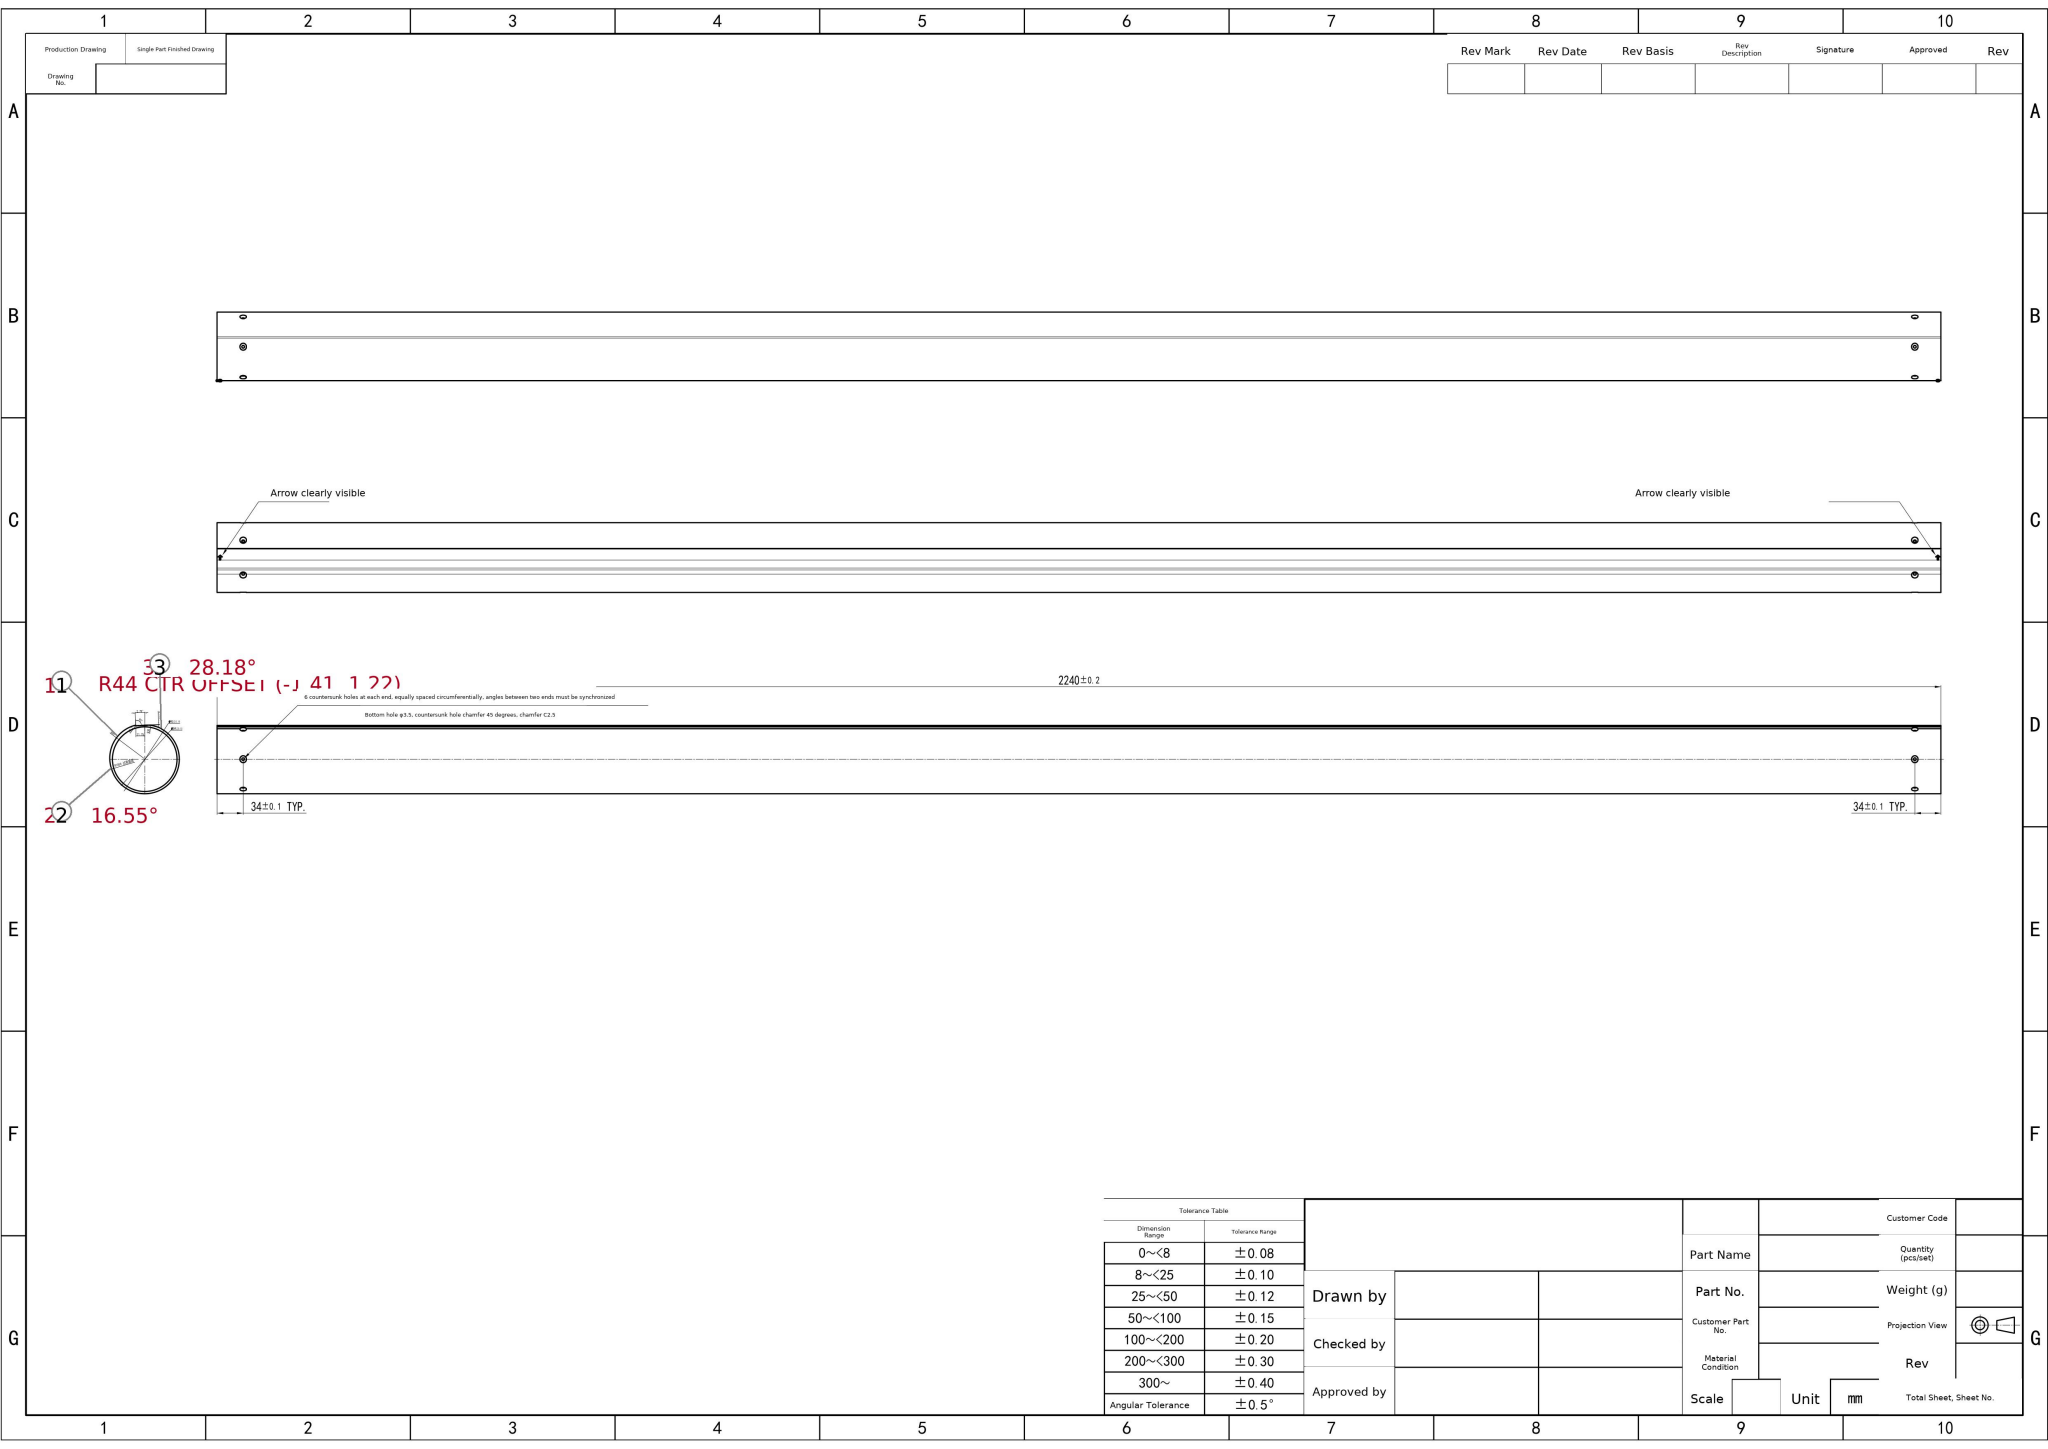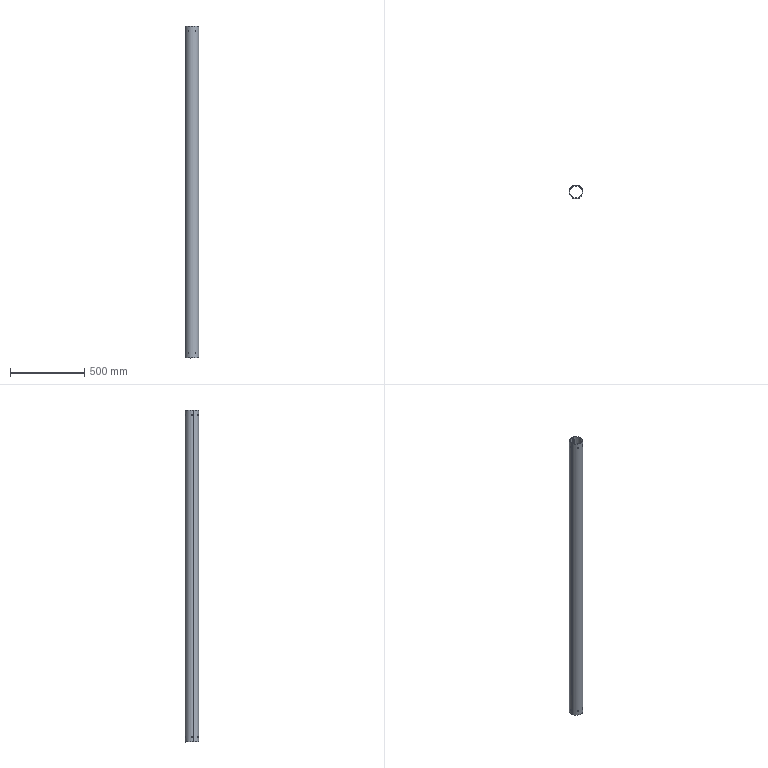Part | SolidWorks | mm | 1 solid | 94 faces | box 90.41 x 88.99 x 2240 mm | volume 1890169 mm3 | cylinder 35 | plane 35 | spline 24 | commonest cylinder face diameters 3.5 x24 84 x2 90 x2 60 x2 87 x2 88 x1 2000 x1 0.4 x1